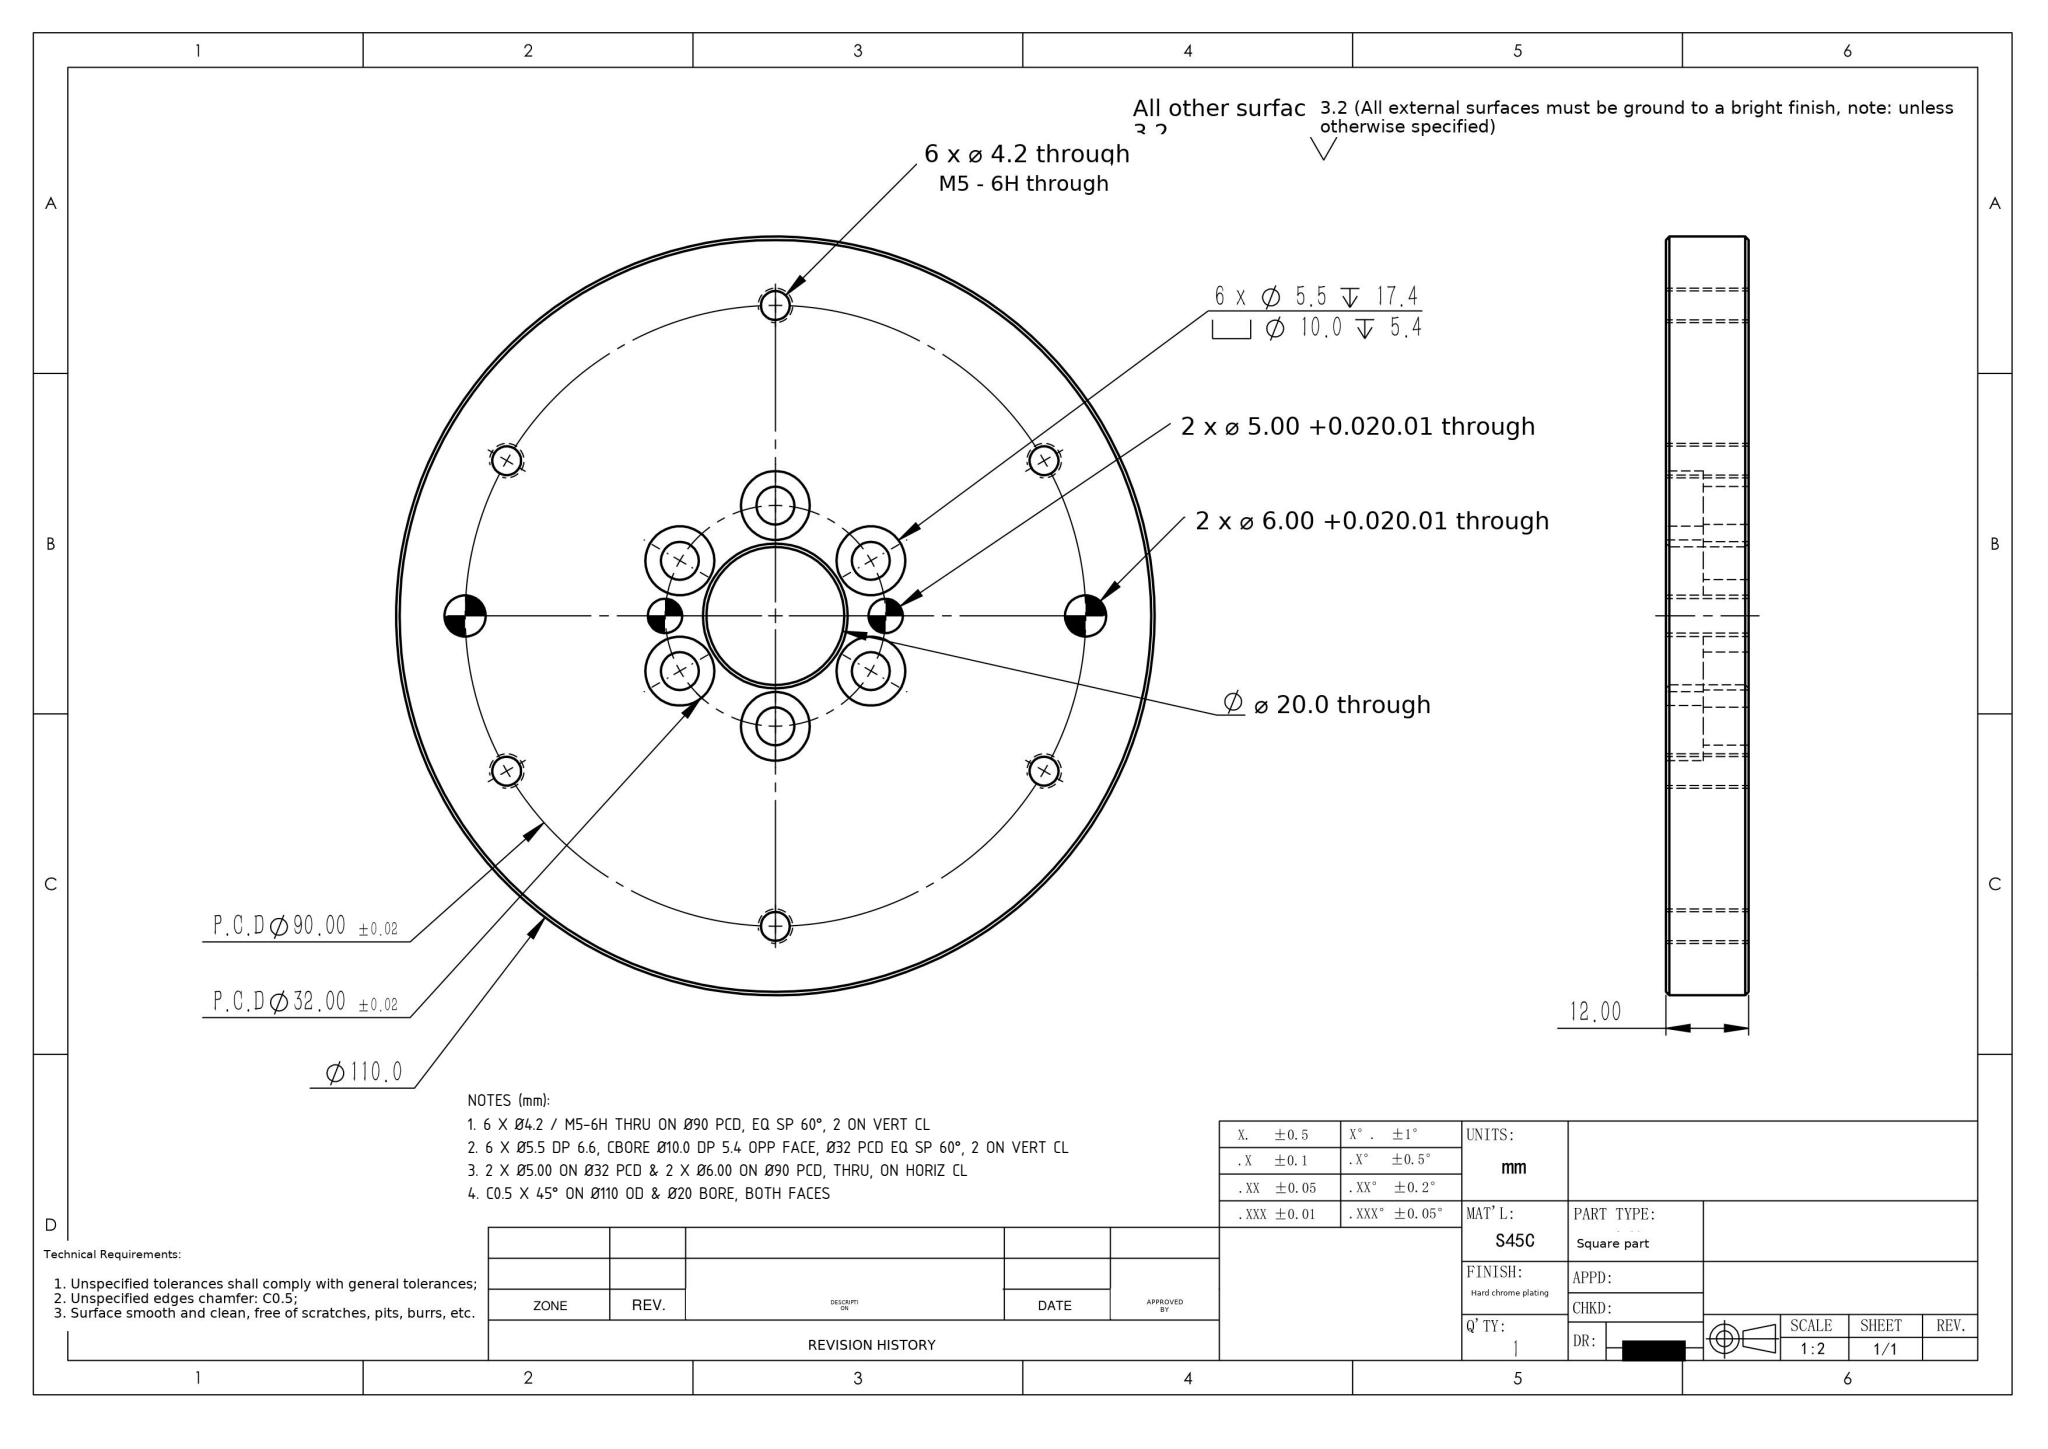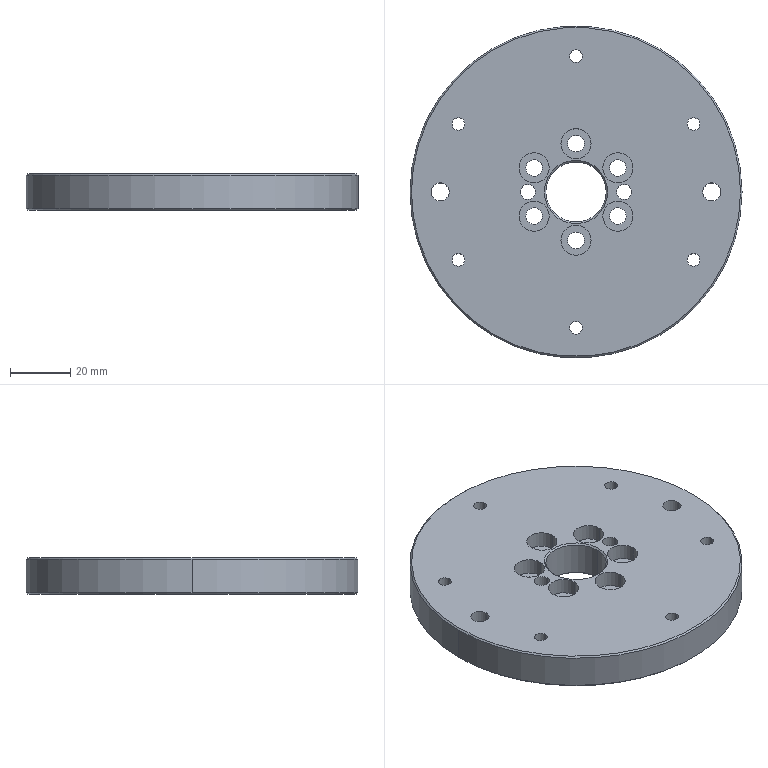Part | SolidWorks | mm | 1 solid | 64 faces | box 110 x 110 x 12 mm | volume 104535 mm3 | cylinder 48 | cone 8 | plane 8 | commonest cylinder face diameters 4.2 x12 10 x12 5.5 x12 5 x4 6 x4 20 x2 110 x2
Drawing notes:
6 X Ø4.2 / M5-6H THRU ON Ø90 PCD, EQ SP 60°, 2 ON VERT CL | from the solid: Ø4.2 thru (L=12.0) at (55,100),(55,10),(93.97,77.5),(16.03,77.5),(16.03,32.5),(93.97,32.5) = R45 from ctr (55,55), 60° spacing
6 X Ø5.5 DP 6.6, CBORE Ø10.0 DP 5.4 OPP FACE, Ø32 PCD EQ SP 60°, 2 ON VERT CL | from the solid: Ø5.5 L=6.6 (z0-6.6) + coaxial Ø10.0 L=5.4 (z6.6-12.0), planes z=0/6.6/12.0; 6 places R16 from ctr at (55,71),(55,39),(68.86,63),(41.14,63),(41.14,47),(68.86,47); sheet 1 DP 17.4 not supported
2 X Ø5.00 ON Ø32 PCD & 2 X Ø6.00 ON Ø90 PCD, THRU, ON HORIZ CL | from the solid: Ø5.0 at (39,55)&(71,55) = R16; Ø6.0 at (10,55)&(100,55) = R45; both pairs on Y=55 CL, L=12.0 thru
C0.5 X 45° ON Ø110 OD & Ø20 BORE, BOTH FACES | from the solid: cones 90° incl at ref Ø109/Ø110 and Ø20/Ø21, 2 each; Ø110 and Ø20 cyl lengths 11.0 of 12.0 thk
build123d program:
from build123d import *

# Parameters (mm, degrees)
SKETCH1_R             = 55
SKETCH1_R_2           = 10
BOSS_EXTRUDE1_DEPTH   = 12
M5_TAPPED_HOLE1_D     = 4.2
CIRPATTERN1_COUNT     = 6
SIZE_MM_DOWEL_HOLE1_D = 6
CHAMFER1_SIZE         = 0.5
SIZE_MM_DOWEL_HOLE2_D = 5


with BuildPart() as part:
    # Sketch1 → Boss-Extrude1 (new body)
    with BuildSketch(Plane.XY):
        Circle(SKETCH1_R)
        Circle(SKETCH1_R_2, mode=Mode.SUBTRACT)
    extrude(amount=BOSS_EXTRUDE1_DEPTH)

    # Sketch3 → M5 Hex Socket Head Cap Screw CBORE1 (revolve, cut)
    with BuildSketch(Plane(origin=(0, 16, 12), x_dir=(0, -1, 0), z_dir=(1, 0, 0))):
        Polygon((0, 0), (0, 19.052), (2.75, 17.4), (2.75, 5.4), (5, 5.4), (5, 0), align=None)
    m5_hex_socket_head_cap_screw_cbore1 = revolve(axis=Axis((0, 16, 18.35), (0, 0, -1)), mode=Mode.SUBTRACT)

    # M5 Tapped Hole1 (through all)
    with Locations(Plane.XY.offset(12)):
        with Locations((0, 45)):
            m5_tapped_hole1 = Hole(M5_TAPPED_HOLE1_D / 2)

    # CirPattern1: M5 Hex Socket Head Cap Screw CBORE1, M5 Tapped Hole1 ×6 about axis
    cirpattern1_axis = Axis((0, 0, 0), (0, 0, 1))
    add([m5_hex_socket_head_cap_screw_cbore1.rotate(cirpattern1_axis, i * 360 / CIRPATTERN1_COUNT) for i in range(1, CIRPATTERN1_COUNT)], mode=Mode.SUBTRACT)
    add([m5_tapped_hole1.rotate(cirpattern1_axis, i * 360 / CIRPATTERN1_COUNT) for i in range(1, CIRPATTERN1_COUNT)], mode=Mode.SUBTRACT)

    # Size mm Dowel Hole1 (through all)
    with Locations(Plane.XY.offset(12)):
        with Locations((-45, 0), (45, 0)):
            Hole(SIZE_MM_DOWEL_HOLE1_D / 2)

    # Chamfer1
    chamfer1_edges = [part.edges().sort_by_distance(p)[0] for p in [
        (-55, 0, 0),
        (-55, 0, 12),
        (-10, 0, 0),
        (-10, 0, 12),
    ]]
    chamfer(chamfer1_edges, length=CHAMFER1_SIZE)

    # Size mm Dowel Hole2 (through all)
    with Locations(Plane.XY.offset(12)):
        with Locations((-16, 0), (16, 0)):
            Hole(SIZE_MM_DOWEL_HOLE2_D / 2)


solid = part.part